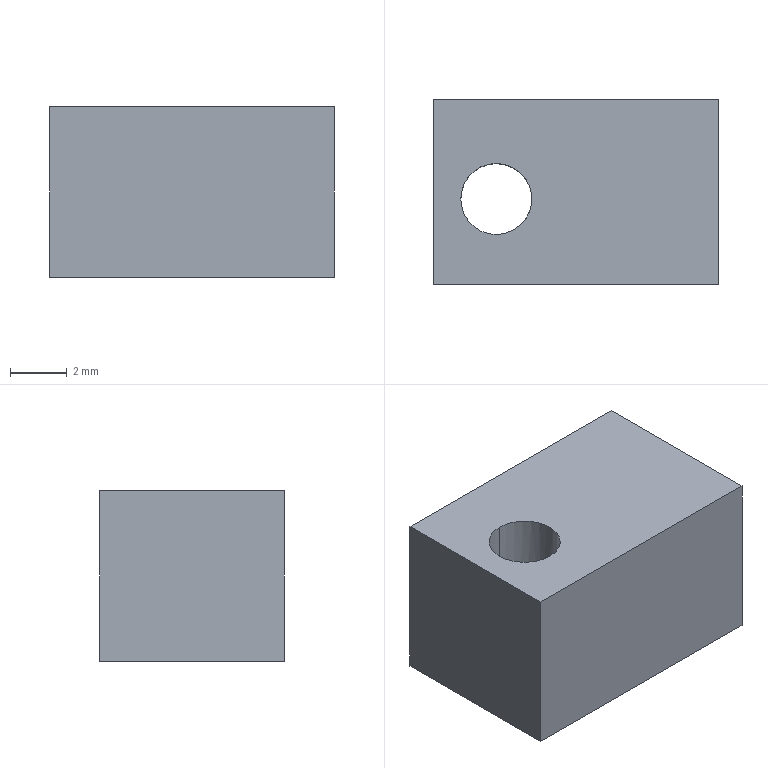CAM job | Mastercam | mm | 8 operations | part box 10 x 6.5 x 6
1. Facing | 24 - 100 平铣刀
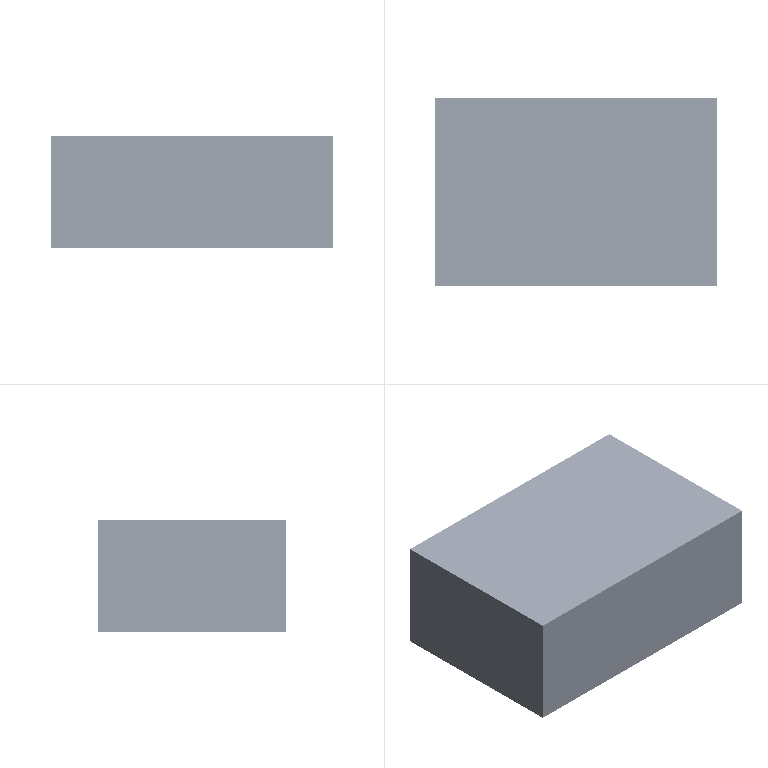2. Contour (Ramp) | 9 - 10 平铣刀
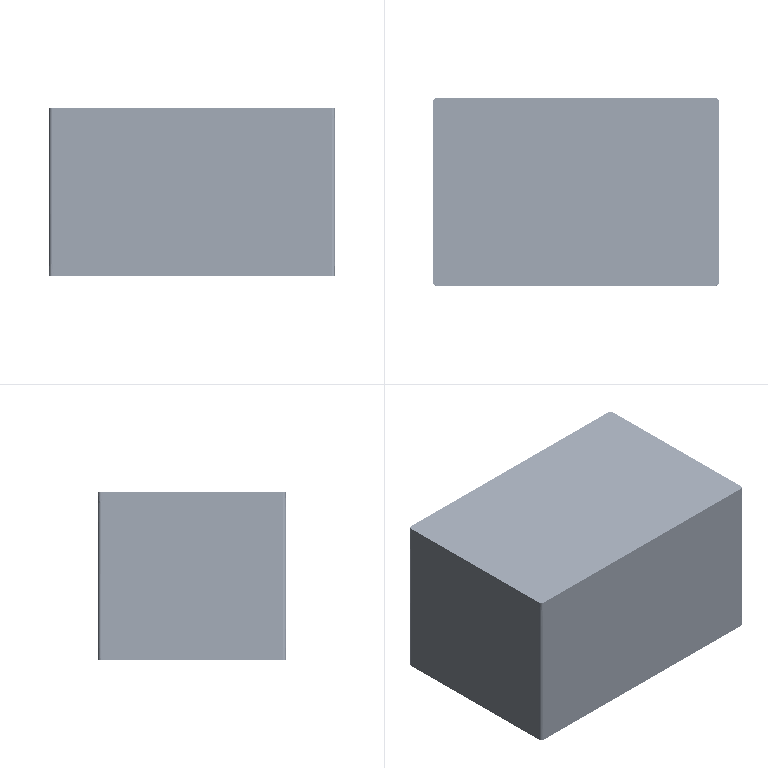3. Contour (2D) | 10 - 10 平铣刀
4. Drill/Counterbore | 5 - 4 倒角刀
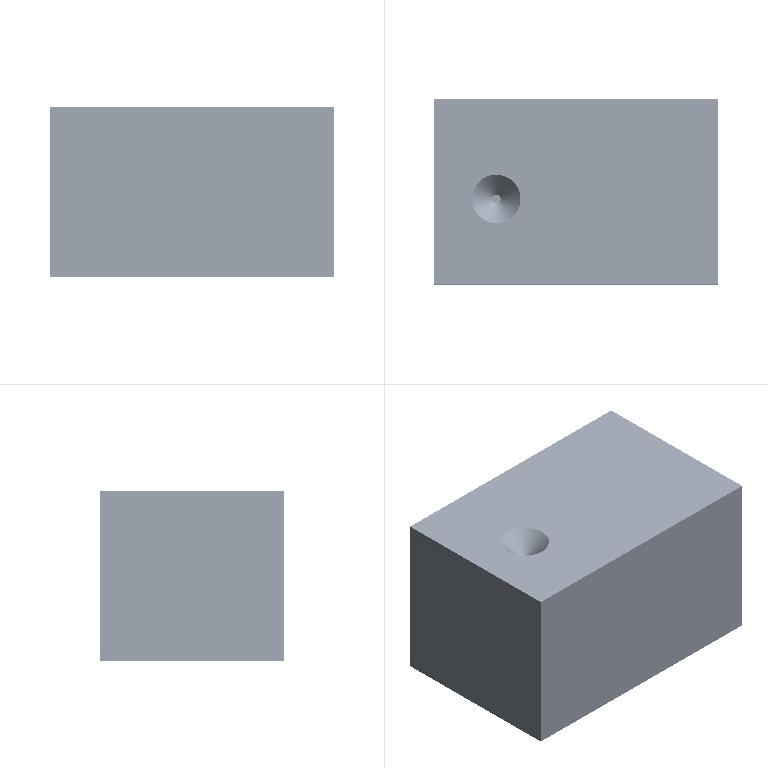5. Contour (2D chamfer) | 5 - 4 倒角刀
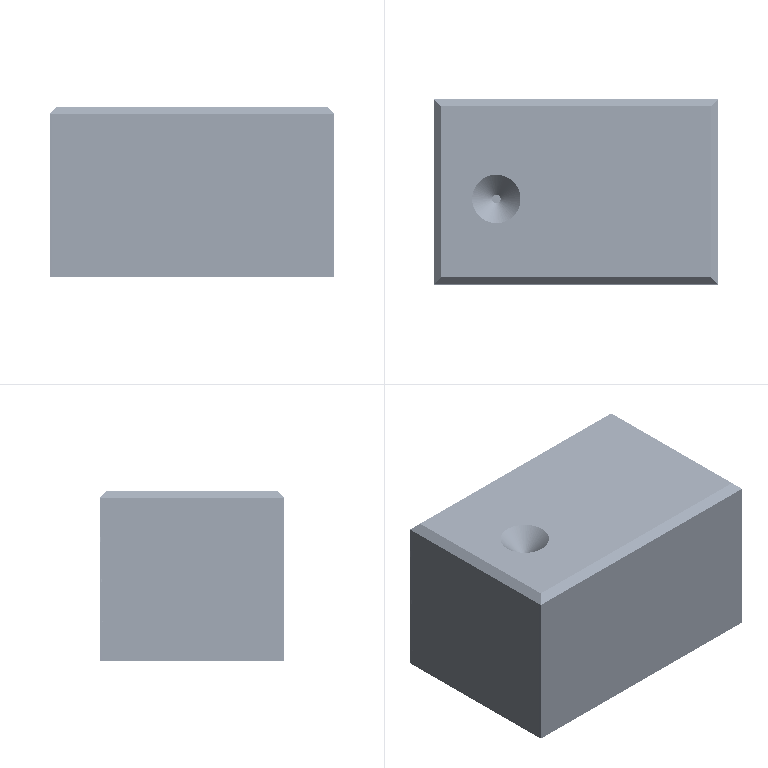6. Facing | 24 - 100 平铣刀
7. Contour (2D chamfer) | 5 - 4 倒角刀
8. Drill/Counterbore | 5 - 4 倒角刀